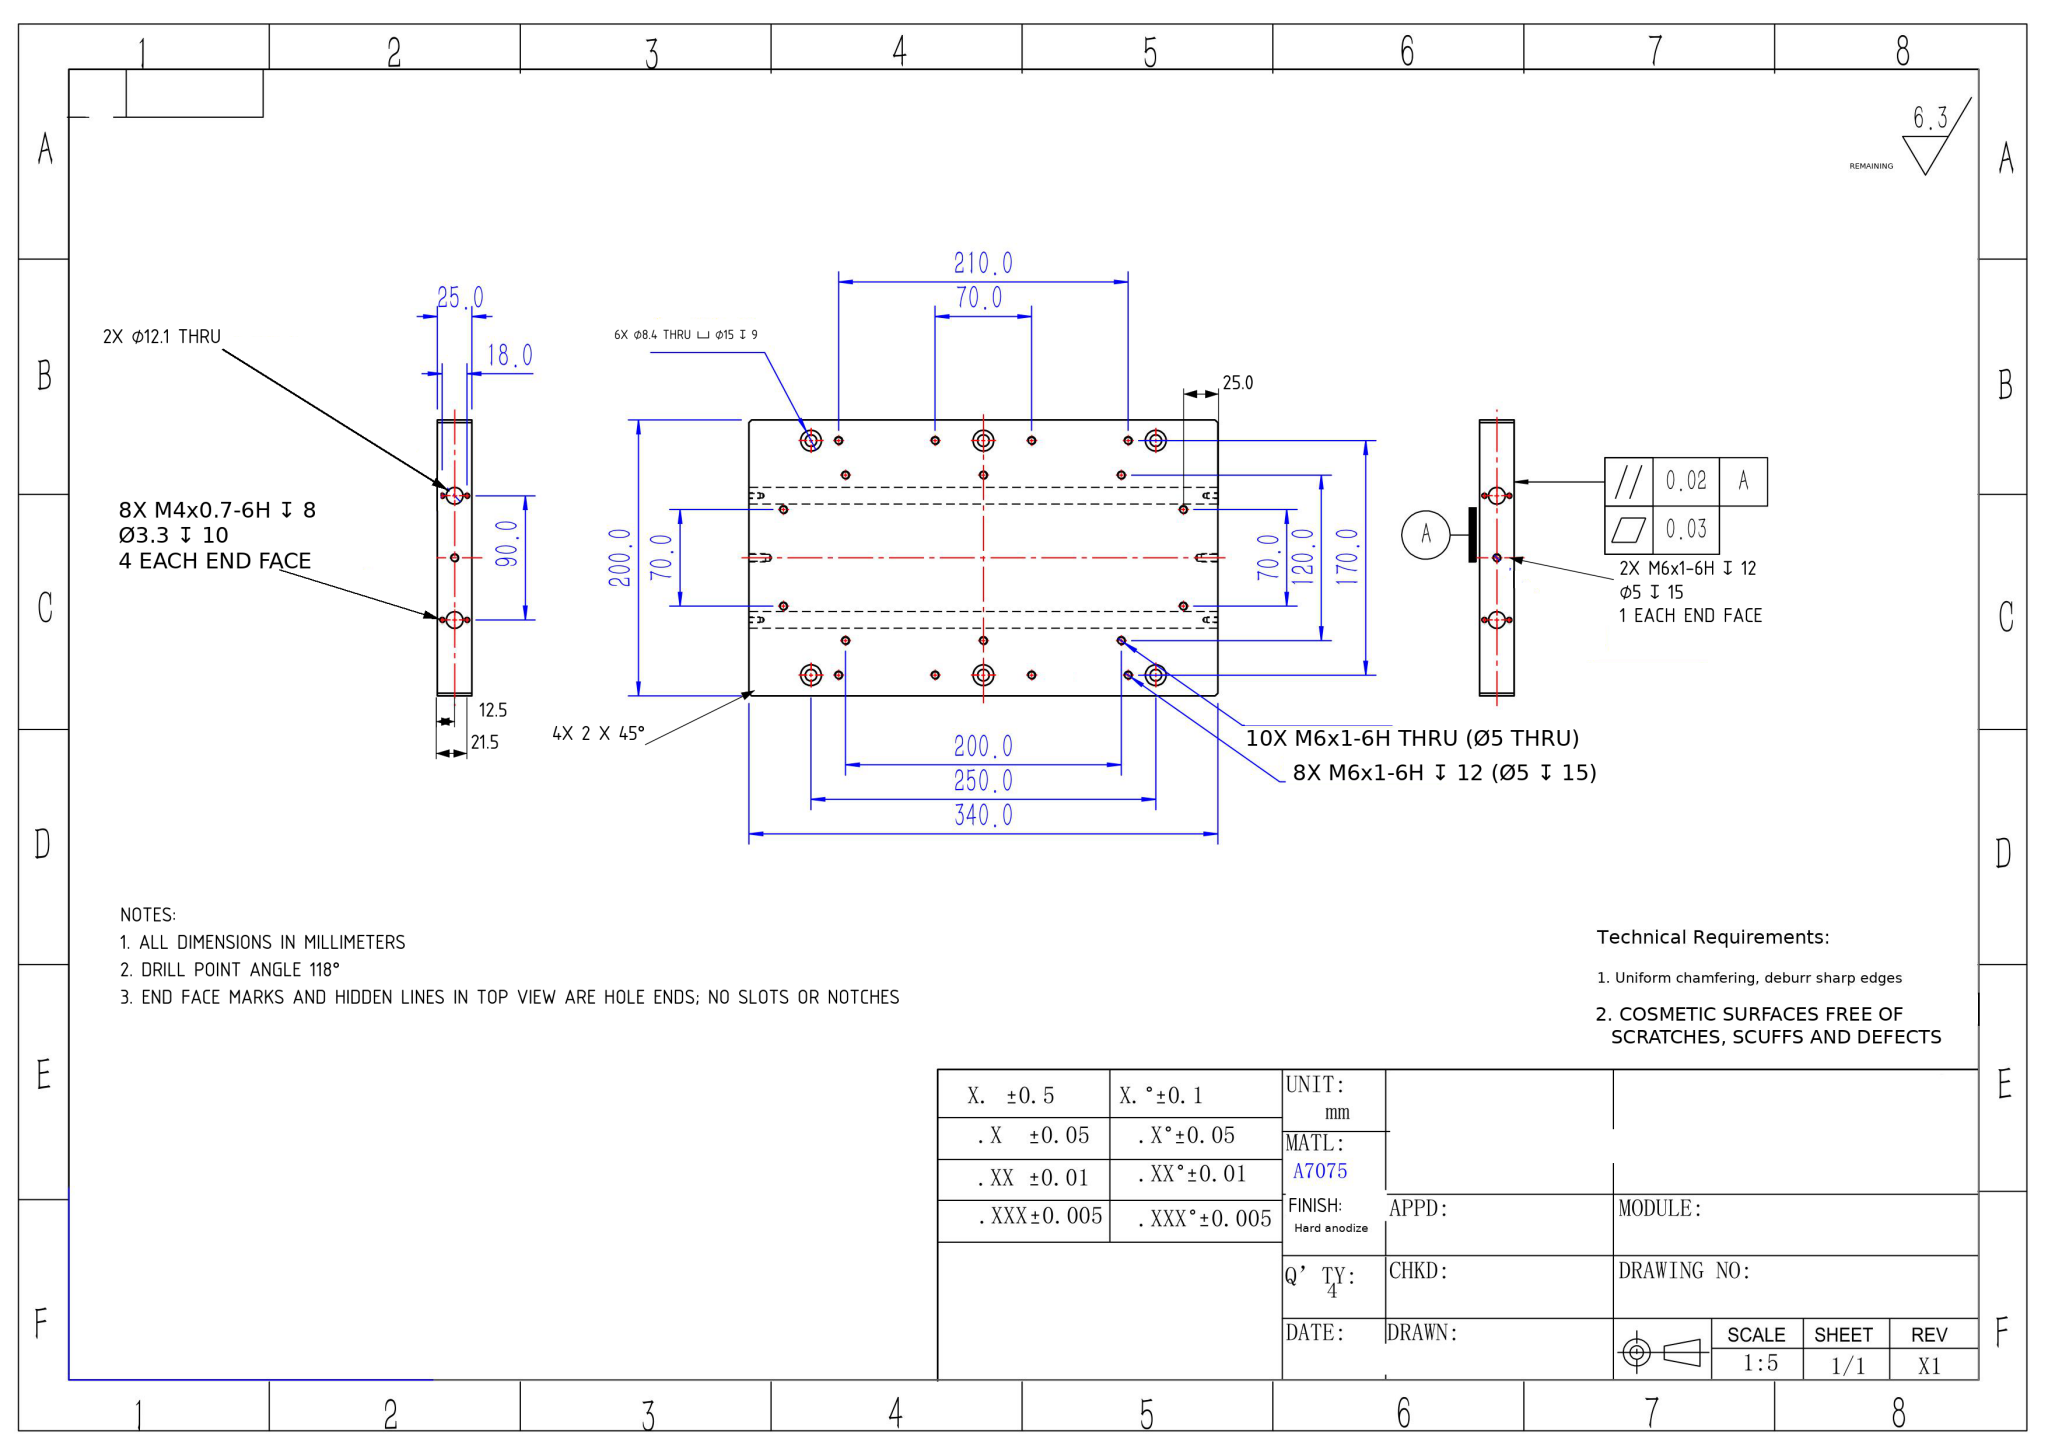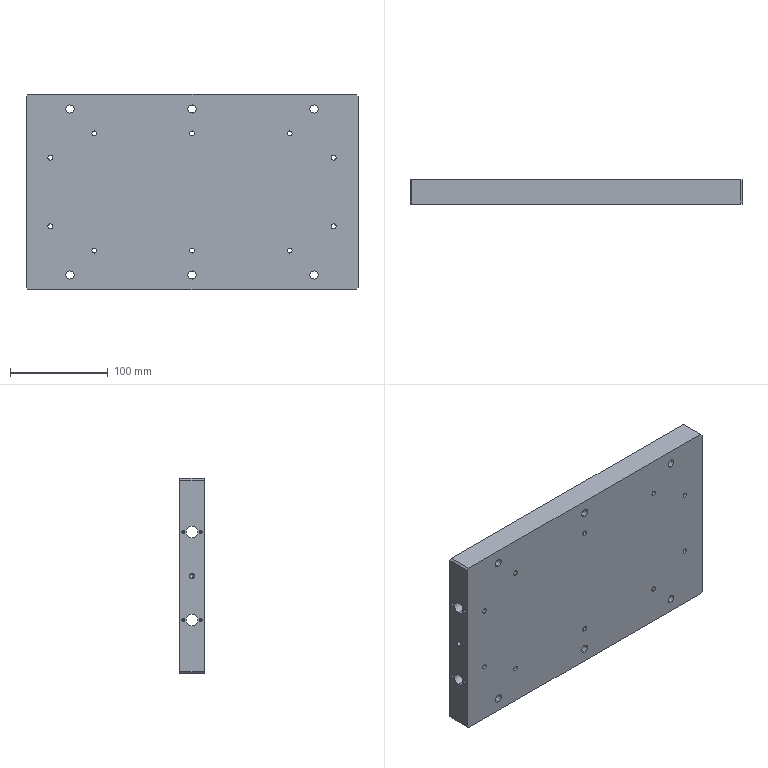Part | NX | mm | 1 solid | 136 faces | box 340 x 25 x 200 mm | volume 1598078 mm3 | cylinder 84 | cone 36 | plane 16 | commonest cylinder face diameters 5 x40 3.3 x16 15 x12 8.4 x12 12.1 x4